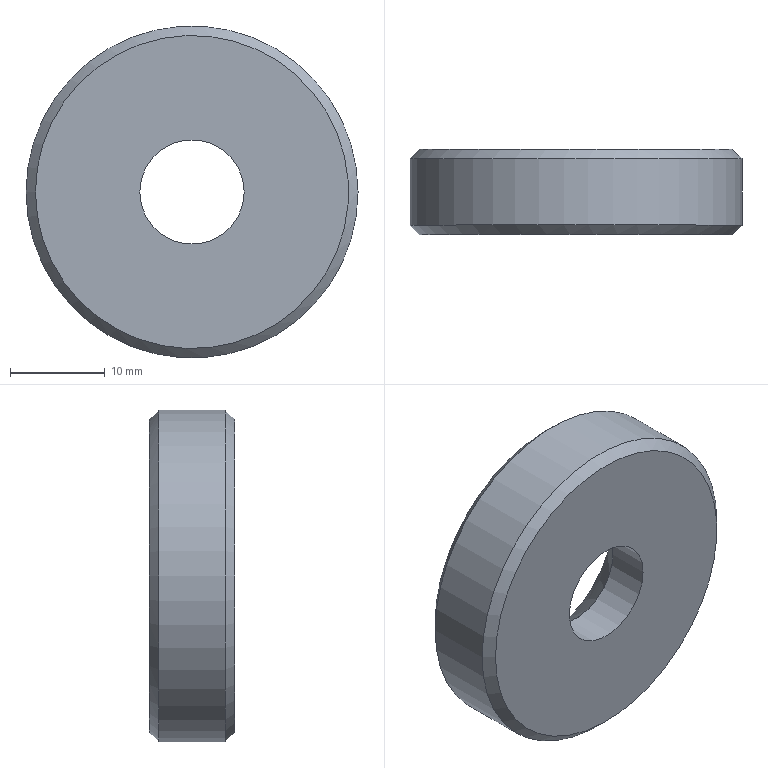Component | NX | END_CAP | 1 solid | 7 faces | box 35 x 9 x 35 mm | volume 7251 mm3 | cone 3 | cylinder 2 | plane 2 | commonest cylinder face diameters 35 x1 11 x1
STEP:
#1=CARTESIAN_POINT('',(0.,0.,0.));
#2=DIRECTION('',(0.,0.,1.));
#3=DIRECTION('',(1.,0.,0.));
#4=AXIS2_PLACEMENT_3D('',#1,#2,#3);
#5=CARTESIAN_POINT('',(-17.5,234.,-0.));
#6=VERTEX_POINT('',#5);
#7=CARTESIAN_POINT('',(0.,234.,-0.));
#8=DIRECTION('',(0.,1.,0.));
#9=DIRECTION('',(-1.,0.,0.));
#10=AXIS2_PLACEMENT_3D('',#7,#8,#9);
#11=CIRCLE('',#10,17.5);
#12=CARTESIAN_POINT('',(0.,242.,-0.));
#13=DIRECTION('',(0.,-1.,0.));
#14=DIRECTION('',(-1.,0.,0.));
#15=AXIS2_PLACEMENT_3D('',#12,#13,#14);
#16=CYLINDRICAL_SURFACE('',#15,17.5);
#17=CARTESIAN_POINT('',(6.283,8.));
#18=DIRECTION('',(-1.,0.));
#19=VECTOR('',#18,1.);
#20=LINE('',#17,#19);
#21=(GEOMETRIC_REPRESENTATION_CONTEXT(2)PARAMETRIC_REPRESENTATION_CONTEXT()REPRESENTATION_CONTEXT('',''));
#22=DEFINITIONAL_REPRESENTATION('',(#20),#21);
#23=PCURVE('',#16,#22);
#24=CARTESIAN_POINT('',(0.,233.,-0.));
#25=DIRECTION('',(0.,1.,0.));
#26=DIRECTION('',(1.,0.,0.));
#27=AXIS2_PLACEMENT_3D('',#24,#25,#26);
#28=CONICAL_SURFACE('',#27,16.5,0.7854);
#29=CARTESIAN_POINT('',(3.142,1.));
#30=DIRECTION('',(1.,0.));
#31=VECTOR('',#30,1.);
#32=LINE('',#29,#31);
#33=(GEOMETRIC_REPRESENTATION_CONTEXT(2)PARAMETRIC_REPRESENTATION_CONTEXT()REPRESENTATION_CONTEXT('',''));
#34=DEFINITIONAL_REPRESENTATION('',(#32),#33);
#35=PCURVE('',#28,#34);
#36=SURFACE_CURVE('',#11,(#23,#35),.PCURVE_S1.);
#37=EDGE_CURVE('',#6,#6,#36,.T.);
#38=ORIENTED_EDGE('',*,*,#37,.T.);
#39=CARTESIAN_POINT('',(-17.5,241.,-0.));
#40=VERTEX_POINT('',#39);
#41=CARTESIAN_POINT('',(-17.5,241.,0.));
#42=CARTESIAN_POINT('',(-17.5,234.,0.));
#43=B_SPLINE_CURVE_WITH_KNOTS('',1,(#41,#42),.UNSPECIFIED.,.F.,.F.,(2,2),(1.,8.),.PIECEWISE_BEZIER_KNOTS.);
#44=CARTESIAN_POINT('',(0.,0.));
#45=DIRECTION('',(0.,1.));
#46=VECTOR('',#45,1.);
#47=LINE('',#44,#46);
#48=(GEOMETRIC_REPRESENTATION_CONTEXT(2)PARAMETRIC_REPRESENTATION_CONTEXT()REPRESENTATION_CONTEXT('',''));
#49=DEFINITIONAL_REPRESENTATION('',(#47),#48);
#50=PCURVE('',#16,#49);
#51=CARTESIAN_POINT('',(6.283,0.));
#52=DIRECTION('',(0.,1.));
#53=VECTOR('',#52,1.);
#54=LINE('',#51,#53);
#55=(GEOMETRIC_REPRESENTATION_CONTEXT(2)PARAMETRIC_REPRESENTATION_CONTEXT()REPRESENTATION_CONTEXT('',''));
#56=DEFINITIONAL_REPRESENTATION('',(#54),#55);
#57=PCURVE('',#16,#56);
#58=SEAM_CURVE('',#43,(#50,#57),.PCURVE_S1.);
#59=EDGE_CURVE('',#40,#6,#58,.T.);
#60=ORIENTED_EDGE('',*,*,#59,.F.);
#61=CARTESIAN_POINT('',(0.,241.,-0.));
#62=DIRECTION('',(0.,-1.,0.));
#63=DIRECTION('',(-1.,0.,0.));
#64=AXIS2_PLACEMENT_3D('',#61,#62,#63);
#65=CIRCLE('',#64,17.5);
#66=CARTESIAN_POINT('',(0.,1.));
#67=DIRECTION('',(1.,0.));
#68=VECTOR('',#67,1.);
#69=LINE('',#66,#68);
#70=(GEOMETRIC_REPRESENTATION_CONTEXT(2)PARAMETRIC_REPRESENTATION_CONTEXT()REPRESENTATION_CONTEXT('',''));
#71=DEFINITIONAL_REPRESENTATION('',(#69),#70);
#72=PCURVE('',#16,#71);
#73=CARTESIAN_POINT('',(0.,241.,-0.));
#74=DIRECTION('',(0.,-1.,0.));
#75=DIRECTION('',(-1.,0.,0.));
#76=AXIS2_PLACEMENT_3D('',#73,#74,#75);
#77=CONICAL_SURFACE('',#76,17.5,0.7854);
#78=CARTESIAN_POINT('',(0.,0.));
#79=DIRECTION('',(1.,0.));
#80=VECTOR('',#79,1.);
#81=LINE('',#78,#80);
#82=(GEOMETRIC_REPRESENTATION_CONTEXT(2)PARAMETRIC_REPRESENTATION_CONTEXT()REPRESENTATION_CONTEXT('',''));
#83=DEFINITIONAL_REPRESENTATION('',(#81),#82);
#84=PCURVE('',#77,#83);
#85=SURFACE_CURVE('',#65,(#72,#84),.PCURVE_S1.);
#86=EDGE_CURVE('',#40,#40,#85,.T.);
#87=ORIENTED_EDGE('',*,*,#86,.T.);
#88=ORIENTED_EDGE('',*,*,#59,.T.);
#89=EDGE_LOOP('',(#38,#60,#87,#88));
#90=FACE_BOUND('',#89,.T.);
#91=ADVANCED_FACE('',(#90),#16,.T.);
#92=CARTESIAN_POINT('',(-16.5,242.,-0.));
#93=VERTEX_POINT('',#92);
#94=CARTESIAN_POINT('',(0.,242.,-0.));
#95=DIRECTION('',(0.,1.,0.));
#96=DIRECTION('',(-1.,0.,0.));
#97=AXIS2_PLACEMENT_3D('',#94,#95,#96);
#98=CIRCLE('',#97,16.5);
#99=CARTESIAN_POINT('',(0.,242.,-0.));
#100=DIRECTION('',(0.,-1.,0.));
#101=DIRECTION('',(-1.,0.,0.));
#102=AXIS2_PLACEMENT_3D('',#99,#100,#101);
#103=PLANE('',#102);
#104=CARTESIAN_POINT('',(16.5,0.));
#105=CARTESIAN_POINT('',(16.5,-28.579));
#106=CARTESIAN_POINT('',(-8.25,-14.289));
#107=CARTESIAN_POINT('',(-33.,-0.));
#108=CARTESIAN_POINT('',(-8.25,14.289));
#109=CARTESIAN_POINT('',(16.5,28.579));
#110=CARTESIAN_POINT('',(16.5,0.));
#111=(BOUNDED_CURVE()B_SPLINE_CURVE(2,(#104,#105,#106,#107,#108,#109,#110),.UNSPECIFIED.,.T.,.F.)B_SPLINE_CURVE_WITH_KNOTS((1,2,2,2,2,1),(-2.094,0.,2.094,4.189,6.283,8.378),.UNSPECIFIED.)CURVE()GEOMETRIC_REPRESENTATION_ITEM()RATIONAL_B_SPLINE_CURVE((1.,0.5,1.,0.5,1.,0.5,1.))REPRESENTATION_ITEM(''));
#112=(GEOMETRIC_REPRESENTATION_CONTEXT(2)PARAMETRIC_REPRESENTATION_CONTEXT()REPRESENTATION_CONTEXT('',''));
#113=DEFINITIONAL_REPRESENTATION('',(#111),#112);
#114=PCURVE('',#103,#113);
#115=CARTESIAN_POINT('',(6.283,-1.));
#116=DIRECTION('',(-1.,0.));
#117=VECTOR('',#116,1.);
#118=LINE('',#115,#117);
#119=(GEOMETRIC_REPRESENTATION_CONTEXT(2)PARAMETRIC_REPRESENTATION_CONTEXT()REPRESENTATION_CONTEXT('',''));
#120=DEFINITIONAL_REPRESENTATION('',(#118),#119);
#121=PCURVE('',#77,#120);
#122=SURFACE_CURVE('',#98,(#114,#121),.PCURVE_S1.);
#123=EDGE_CURVE('',#93,#93,#122,.T.);
#124=ORIENTED_EDGE('',*,*,#123,.T.);
#125=EDGE_LOOP('',(#124));
#126=FACE_BOUND('',#125,.T.);
#127=CARTESIAN_POINT('',(-10.,242.,-0.));
#128=VERTEX_POINT('',#127);
#129=CARTESIAN_POINT('',(0.,242.,-0.));
#130=DIRECTION('',(0.,-1.,0.));
#131=DIRECTION('',(-1.,0.,0.));
#132=AXIS2_PLACEMENT_3D('',#129,#130,#131);
#133=CIRCLE('',#132,10.);
#134=CARTESIAN_POINT('',(0.,0.));
#135=DIRECTION('',(1.,0.));
#136=AXIS2_PLACEMENT_2D('',#134,#135);
#137=CIRCLE('',#136,10.);
#138=(GEOMETRIC_REPRESENTATION_CONTEXT(2)PARAMETRIC_REPRESENTATION_CONTEXT()REPRESENTATION_CONTEXT('',''));
#139=DEFINITIONAL_REPRESENTATION('',(#137),#138);
#140=PCURVE('',#103,#139);
#141=CARTESIAN_POINT('',(0.,242.,-0.));
#142=DIRECTION('',(0.,1.,0.));
#143=DIRECTION('',(1.,0.,0.));
#144=AXIS2_PLACEMENT_3D('',#141,#142,#143);
#145=CONICAL_SURFACE('',#144,10.,0.7854);
#146=CARTESIAN_POINT('',(9.425,0.));
#147=DIRECTION('',(-1.,0.));
#148=VECTOR('',#147,1.);
#149=LINE('',#146,#148);
#150=(GEOMETRIC_REPRESENTATION_CONTEXT(2)PARAMETRIC_REPRESENTATION_CONTEXT()REPRESENTATION_CONTEXT('',''));
#151=DEFINITIONAL_REPRESENTATION('',(#149),#150);
#152=PCURVE('',#145,#151);
#153=SURFACE_CURVE('',#133,(#140,#152),.PCURVE_S1.);
#154=EDGE_CURVE('',#128,#128,#153,.T.);
#155=ORIENTED_EDGE('',*,*,#154,.T.);
#156=EDGE_LOOP('',(#155));
#157=FACE_BOUND('',#156,.T.);
#158=ADVANCED_FACE('',(#126,#157),#103,.F.);
#159=CARTESIAN_POINT('',(-16.5,233.,-0.));
#160=VERTEX_POINT('',#159);
#161=CARTESIAN_POINT('',(0.,233.,-0.));
#162=DIRECTION('',(0.,-1.,0.));
#163=DIRECTION('',(-1.,0.,0.));
#164=AXIS2_PLACEMENT_3D('',#161,#162,#163);
#165=CIRCLE('',#164,16.5);
#166=CARTESIAN_POINT('',(0.,233.,-0.));
#167=DIRECTION('',(0.,-1.,0.));
#168=DIRECTION('',(-1.,0.,0.));
#169=AXIS2_PLACEMENT_3D('',#166,#167,#168);
#170=PLANE('',#169);
#171=CARTESIAN_POINT('',(0.,0.));
#172=DIRECTION('',(1.,0.));
#173=AXIS2_PLACEMENT_2D('',#171,#172);
#174=CIRCLE('',#173,16.5);
#175=(GEOMETRIC_REPRESENTATION_CONTEXT(2)PARAMETRIC_REPRESENTATION_CONTEXT()REPRESENTATION_CONTEXT('',''));
#176=DEFINITIONAL_REPRESENTATION('',(#174),#175);
#177=PCURVE('',#170,#176);
#178=CARTESIAN_POINT('',(9.425,0.));
#179=DIRECTION('',(-1.,0.));
#180=VECTOR('',#179,1.);
#181=LINE('',#178,#180);
#182=(GEOMETRIC_REPRESENTATION_CONTEXT(2)PARAMETRIC_REPRESENTATION_CONTEXT()REPRESENTATION_CONTEXT('',''));
#183=DEFINITIONAL_REPRESENTATION('',(#181),#182);
#184=PCURVE('',#28,#183);
#185=SURFACE_CURVE('',#165,(#177,#184),.PCURVE_S1.);
#186=EDGE_CURVE('',#160,#160,#185,.T.);
#187=ORIENTED_EDGE('',*,*,#186,.T.);
#188=EDGE_LOOP('',(#187));
#189=FACE_BOUND('',#188,.T.);
#190=CARTESIAN_POINT('',(-5.5,233.,-0.));
#191=VERTEX_POINT('',#190);
#192=CARTESIAN_POINT('',(0.,233.,-0.));
#193=DIRECTION('',(0.,-1.,0.));
#194=DIRECTION('',(-1.,0.,0.));
#195=AXIS2_PLACEMENT_3D('',#192,#193,#194);
#196=CIRCLE('',#195,5.5);
#197=CARTESIAN_POINT('',(0.,0.));
#198=DIRECTION('',(1.,0.));
#199=AXIS2_PLACEMENT_2D('',#197,#198);
#200=CIRCLE('',#199,5.5);
#201=(GEOMETRIC_REPRESENTATION_CONTEXT(2)PARAMETRIC_REPRESENTATION_CONTEXT()REPRESENTATION_CONTEXT('',''));
#202=DEFINITIONAL_REPRESENTATION('',(#200),#201);
#203=PCURVE('',#170,#202);
#204=CARTESIAN_POINT('',(0.,233.,-0.));
#205=DIRECTION('',(0.,-1.,0.));
#206=DIRECTION('',(-1.,0.,0.));
#207=AXIS2_PLACEMENT_3D('',#204,#205,#206);
#208=CYLINDRICAL_SURFACE('',#207,5.5);
#209=CARTESIAN_POINT('',(0.,0.));
#210=DIRECTION('',(1.,0.));
#211=VECTOR('',#210,1.);
#212=LINE('',#209,#211);
#213=(GEOMETRIC_REPRESENTATION_CONTEXT(2)PARAMETRIC_REPRESENTATION_CONTEXT()REPRESENTATION_CONTEXT('',''));
#214=DEFINITIONAL_REPRESENTATION('',(#212),#213);
#215=PCURVE('',#208,#214);
#216=SURFACE_CURVE('',#196,(#203,#215),.PCURVE_S1.);
#217=EDGE_CURVE('',#191,#191,#216,.T.);
#218=ORIENTED_EDGE('',*,*,#217,.F.);
#219=EDGE_LOOP('',(#218));
#220=FACE_BOUND('',#219,.T.);
#221=ADVANCED_FACE('',(#189,#220),#170,.T.);
#222=CARTESIAN_POINT('',(-5.5,237.5,-0.));
#223=VERTEX_POINT('',#222);
#224=CARTESIAN_POINT('',(0.,237.5,-0.));
#225=DIRECTION('',(0.,1.,0.));
#226=DIRECTION('',(-1.,0.,0.));
#227=AXIS2_PLACEMENT_3D('',#224,#225,#226);
#228=CIRCLE('',#227,5.5);
#229=CARTESIAN_POINT('',(3.142,-4.5));
#230=DIRECTION('',(1.,0.));
#231=VECTOR('',#230,1.);
#232=LINE('',#229,#231);
#233=(GEOMETRIC_REPRESENTATION_CONTEXT(2)PARAMETRIC_REPRESENTATION_CONTEXT()REPRESENTATION_CONTEXT('',''));
#234=DEFINITIONAL_REPRESENTATION('',(#232),#233);
#235=PCURVE('',#145,#234);
#236=CARTESIAN_POINT('',(6.283,-4.5));
#237=DIRECTION('',(-1.,0.));
#238=VECTOR('',#237,1.);
#239=LINE('',#236,#238);
#240=(GEOMETRIC_REPRESENTATION_CONTEXT(2)PARAMETRIC_REPRESENTATION_CONTEXT()REPRESENTATION_CONTEXT('',''));
#241=DEFINITIONAL_REPRESENTATION('',(#239),#240);
#242=PCURVE('',#208,#241);
#243=SURFACE_CURVE('',#228,(#235,#242),.PCURVE_S1.);
#244=EDGE_CURVE('',#223,#223,#243,.T.);
#245=ORIENTED_EDGE('',*,*,#244,.T.);
#246=CARTESIAN_POINT('',(-5.5,237.5,-0.));
#247=CARTESIAN_POINT('',(-10.,242.,-0.));
#248=B_SPLINE_CURVE_WITH_KNOTS('',1,(#246,#247),.UNSPECIFIED.,.F.,.F.,(2,2),(-6.364,0.),.PIECEWISE_BEZIER_KNOTS.);
#249=CARTESIAN_POINT('',(9.425,0.));
#250=DIRECTION('',(0.,1.));
#251=VECTOR('',#250,1.);
#252=LINE('',#249,#251);
#253=(GEOMETRIC_REPRESENTATION_CONTEXT(2)PARAMETRIC_REPRESENTATION_CONTEXT()REPRESENTATION_CONTEXT('',''));
#254=DEFINITIONAL_REPRESENTATION('',(#252),#253);
#255=PCURVE('',#145,#254);
#256=CARTESIAN_POINT('',(3.142,0.));
#257=DIRECTION('',(0.,1.));
#258=VECTOR('',#257,1.);
#259=LINE('',#256,#258);
#260=(GEOMETRIC_REPRESENTATION_CONTEXT(2)PARAMETRIC_REPRESENTATION_CONTEXT()REPRESENTATION_CONTEXT('',''));
#261=DEFINITIONAL_REPRESENTATION('',(#259),#260);
#262=PCURVE('',#145,#261);
#263=SEAM_CURVE('',#248,(#255,#262),.PCURVE_S1.);
#264=EDGE_CURVE('',#223,#128,#263,.T.);
#265=ORIENTED_EDGE('',*,*,#264,.T.);
#266=ORIENTED_EDGE('',*,*,#154,.T.);
#267=ORIENTED_EDGE('',*,*,#264,.F.);
#268=EDGE_LOOP('',(#245,#265,#266,#267));
#269=FACE_BOUND('',#268,.F.);
#270=ADVANCED_FACE('',(#269),#145,.F.);
#271=ORIENTED_EDGE('',*,*,#217,.F.);
#272=CARTESIAN_POINT('',(-5.5,237.5,0.));
#273=CARTESIAN_POINT('',(-5.5,233.,0.));
#274=B_SPLINE_CURVE_WITH_KNOTS('',1,(#272,#273),.UNSPECIFIED.,.F.,.F.,(2,2),(-4.5,0.),.PIECEWISE_BEZIER_KNOTS.);
#275=CARTESIAN_POINT('',(0.,0.));
#276=DIRECTION('',(0.,1.));
#277=VECTOR('',#276,1.);
#278=LINE('',#275,#277);
#279=(GEOMETRIC_REPRESENTATION_CONTEXT(2)PARAMETRIC_REPRESENTATION_CONTEXT()REPRESENTATION_CONTEXT('',''));
#280=DEFINITIONAL_REPRESENTATION('',(#278),#279);
#281=PCURVE('',#208,#280);
#282=CARTESIAN_POINT('',(6.283,0.));
#283=DIRECTION('',(0.,1.));
#284=VECTOR('',#283,1.);
#285=LINE('',#282,#284);
#286=(GEOMETRIC_REPRESENTATION_CONTEXT(2)PARAMETRIC_REPRESENTATION_CONTEXT()REPRESENTATION_CONTEXT('',''));
#287=DEFINITIONAL_REPRESENTATION('',(#285),#286);
#288=PCURVE('',#208,#287);
#289=SEAM_CURVE('',#274,(#281,#288),.PCURVE_S1.);
#290=EDGE_CURVE('',#223,#191,#289,.T.);
#291=ORIENTED_EDGE('',*,*,#290,.F.);
#292=ORIENTED_EDGE('',*,*,#244,.F.);
#293=ORIENTED_EDGE('',*,*,#290,.T.);
#294=EDGE_LOOP('',(#271,#291,#292,#293));
#295=FACE_BOUND('',#294,.F.);
#296=ADVANCED_FACE('',(#295),#208,.F.);
#297=ORIENTED_EDGE('',*,*,#37,.F.);
#298=CARTESIAN_POINT('',(-16.5,233.,-0.));
#299=CARTESIAN_POINT('',(-17.5,234.,-0.));
#300=B_SPLINE_CURVE_WITH_KNOTS('',1,(#298,#299),.UNSPECIFIED.,.F.,.F.,(2,2),(0.,1.414),.PIECEWISE_BEZIER_KNOTS.);
#301=CARTESIAN_POINT('',(3.142,0.));
#302=DIRECTION('',(0.,1.));
#303=VECTOR('',#302,1.);
#304=LINE('',#301,#303);
#305=(GEOMETRIC_REPRESENTATION_CONTEXT(2)PARAMETRIC_REPRESENTATION_CONTEXT()REPRESENTATION_CONTEXT('',''));
#306=DEFINITIONAL_REPRESENTATION('',(#304),#305);
#307=PCURVE('',#28,#306);
#308=CARTESIAN_POINT('',(9.425,0.));
#309=DIRECTION('',(0.,1.));
#310=VECTOR('',#309,1.);
#311=LINE('',#308,#310);
#312=(GEOMETRIC_REPRESENTATION_CONTEXT(2)PARAMETRIC_REPRESENTATION_CONTEXT()REPRESENTATION_CONTEXT('',''));
#313=DEFINITIONAL_REPRESENTATION('',(#311),#312);
#314=PCURVE('',#28,#313);
#315=SEAM_CURVE('',#300,(#307,#314),.PCURVE_S1.);
#316=EDGE_CURVE('',#160,#6,#315,.T.);
#317=ORIENTED_EDGE('',*,*,#316,.F.);
#318=ORIENTED_EDGE('',*,*,#186,.F.);
#319=ORIENTED_EDGE('',*,*,#316,.T.);
#320=EDGE_LOOP('',(#297,#317,#318,#319));
#321=FACE_BOUND('',#320,.T.);
#322=ADVANCED_FACE('',(#321),#28,.T.);
#323=ORIENTED_EDGE('',*,*,#123,.F.);
#324=CARTESIAN_POINT('',(-16.5,242.,-0.));
#325=CARTESIAN_POINT('',(-17.5,241.,-0.));
#326=B_SPLINE_CURVE_WITH_KNOTS('',1,(#324,#325),.UNSPECIFIED.,.F.,.F.,(2,2),(-1.414,0.),.PIECEWISE_BEZIER_KNOTS.);
#327=CARTESIAN_POINT('',(6.283,0.));
#328=DIRECTION('',(0.,1.));
#329=VECTOR('',#328,1.);
#330=LINE('',#327,#329);
#331=(GEOMETRIC_REPRESENTATION_CONTEXT(2)PARAMETRIC_REPRESENTATION_CONTEXT()REPRESENTATION_CONTEXT('',''));
#332=DEFINITIONAL_REPRESENTATION('',(#330),#331);
#333=PCURVE('',#77,#332);
#334=CARTESIAN_POINT('',(0.,0.));
#335=DIRECTION('',(0.,1.));
#336=VECTOR('',#335,1.);
#337=LINE('',#334,#336);
#338=(GEOMETRIC_REPRESENTATION_CONTEXT(2)PARAMETRIC_REPRESENTATION_CONTEXT()REPRESENTATION_CONTEXT('',''));
#339=DEFINITIONAL_REPRESENTATION('',(#337),#338);
#340=PCURVE('',#77,#339);
#341=SEAM_CURVE('',#326,(#333,#340),.PCURVE_S1.);
#342=EDGE_CURVE('',#93,#40,#341,.T.);
#343=ORIENTED_EDGE('',*,*,#342,.T.);
#344=ORIENTED_EDGE('',*,*,#86,.F.);
#345=ORIENTED_EDGE('',*,*,#342,.F.);
#346=EDGE_LOOP('',(#323,#343,#344,#345));
#347=FACE_BOUND('',#346,.T.);
#348=ADVANCED_FACE('',(#347),#77,.T.);
#349=CLOSED_SHELL('',(#91,#158,#221,#270,#296,#322,#348));
#350=MANIFOLD_SOLID_BREP('',#349);
#351=(LENGTH_UNIT()NAMED_UNIT(*)SI_UNIT(.MILLI.,.METRE.));
#352=UNCERTAINTY_MEASURE_WITH_UNIT(LENGTH_MEASURE(0.00001),#351,'','');
#353=(NAMED_UNIT(*)PLANE_ANGLE_UNIT()SI_UNIT($,.RADIAN.));
#354=(NAMED_UNIT(*)SI_UNIT($,.STERADIAN.)SOLID_ANGLE_UNIT());
#355=(GEOMETRIC_REPRESENTATION_CONTEXT(3)GLOBAL_UNCERTAINTY_ASSIGNED_CONTEXT((#352))GLOBAL_UNIT_ASSIGNED_CONTEXT((#351,#353,#354))REPRESENTATION_CONTEXT('',''));
#356=ADVANCED_BREP_SHAPE_REPRESENTATION('',(#4,#350),#355);